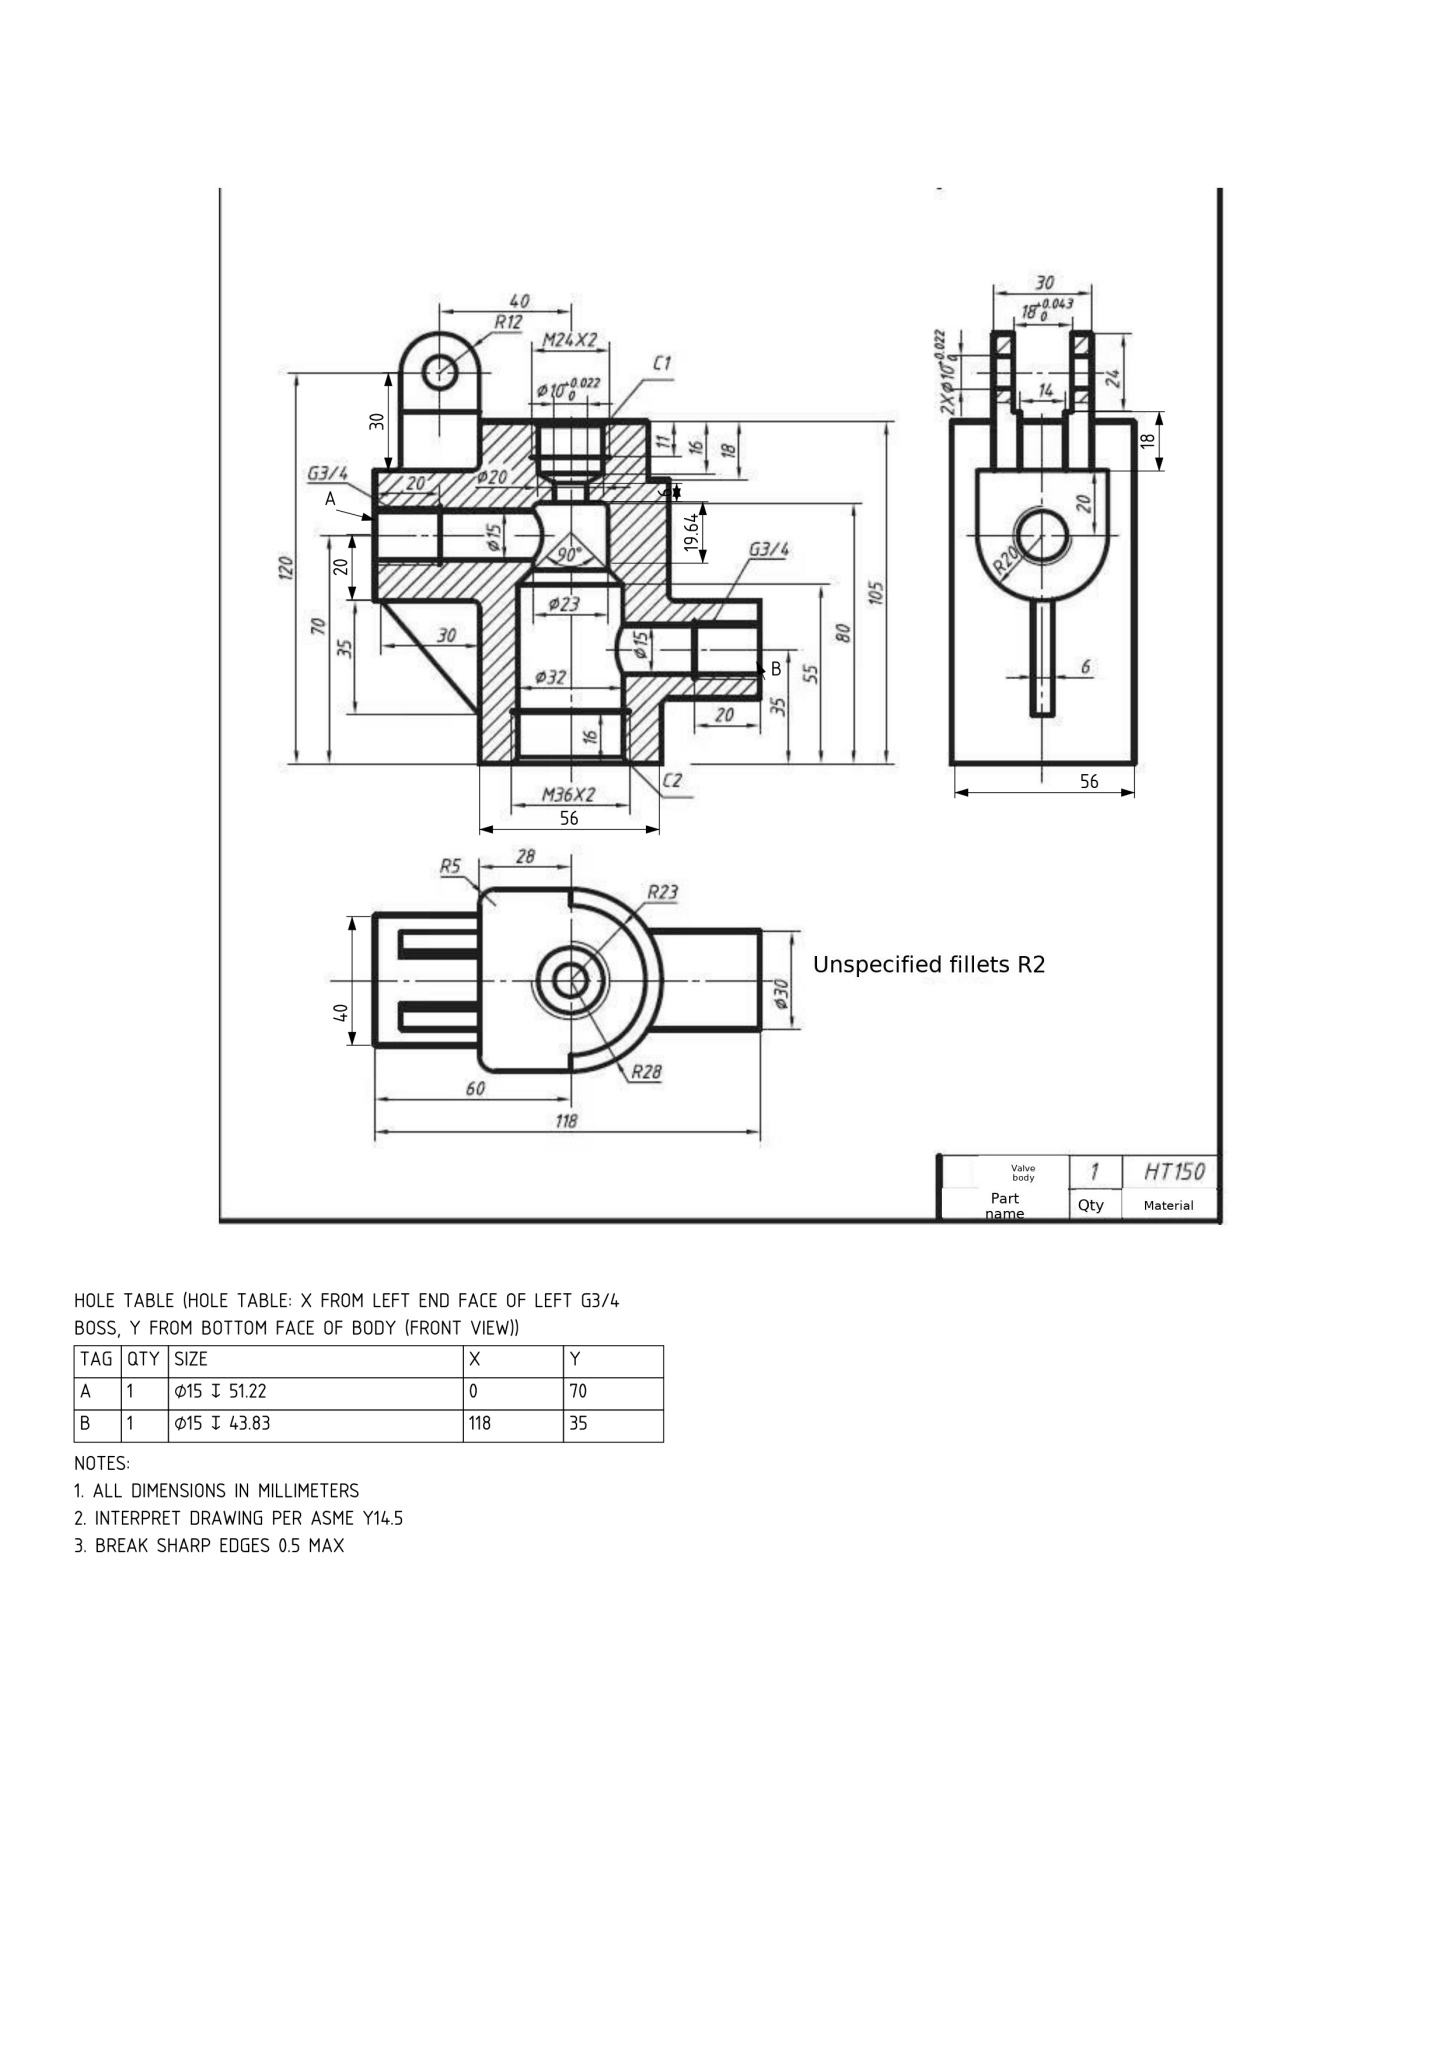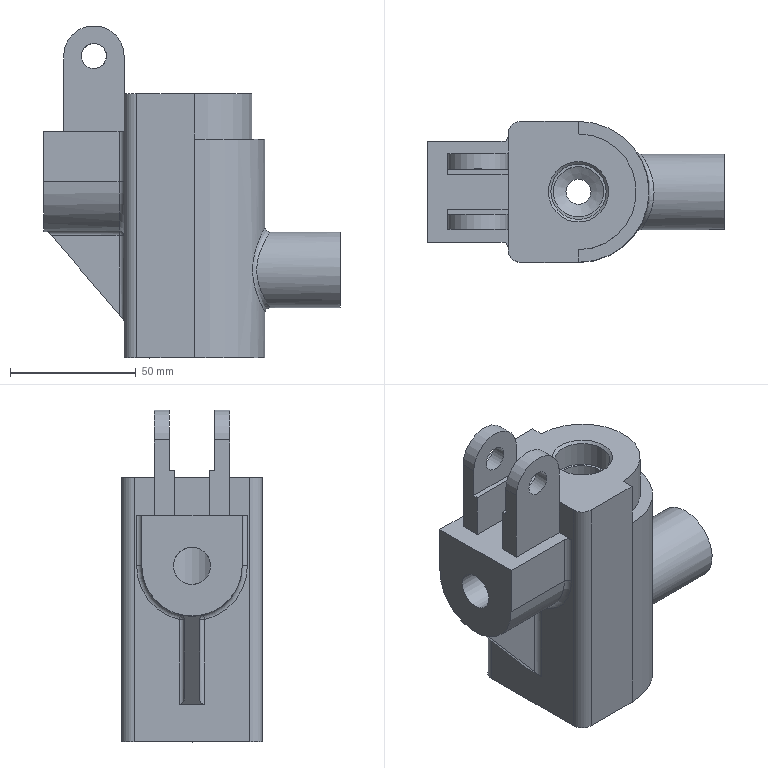Part | NX | mm | 1 solid | 65 faces | box 118 x 56 x 132 mm | volume 288896 mm3 | plane 32 | cylinder 24 | cone 4 | torus 2 | sphere 2 | spline 1 | commonest cylinder face diameters 4 x6 10 x5 24 x2 14.797 x2 56 x1 40 x1 30 x1 34 x1